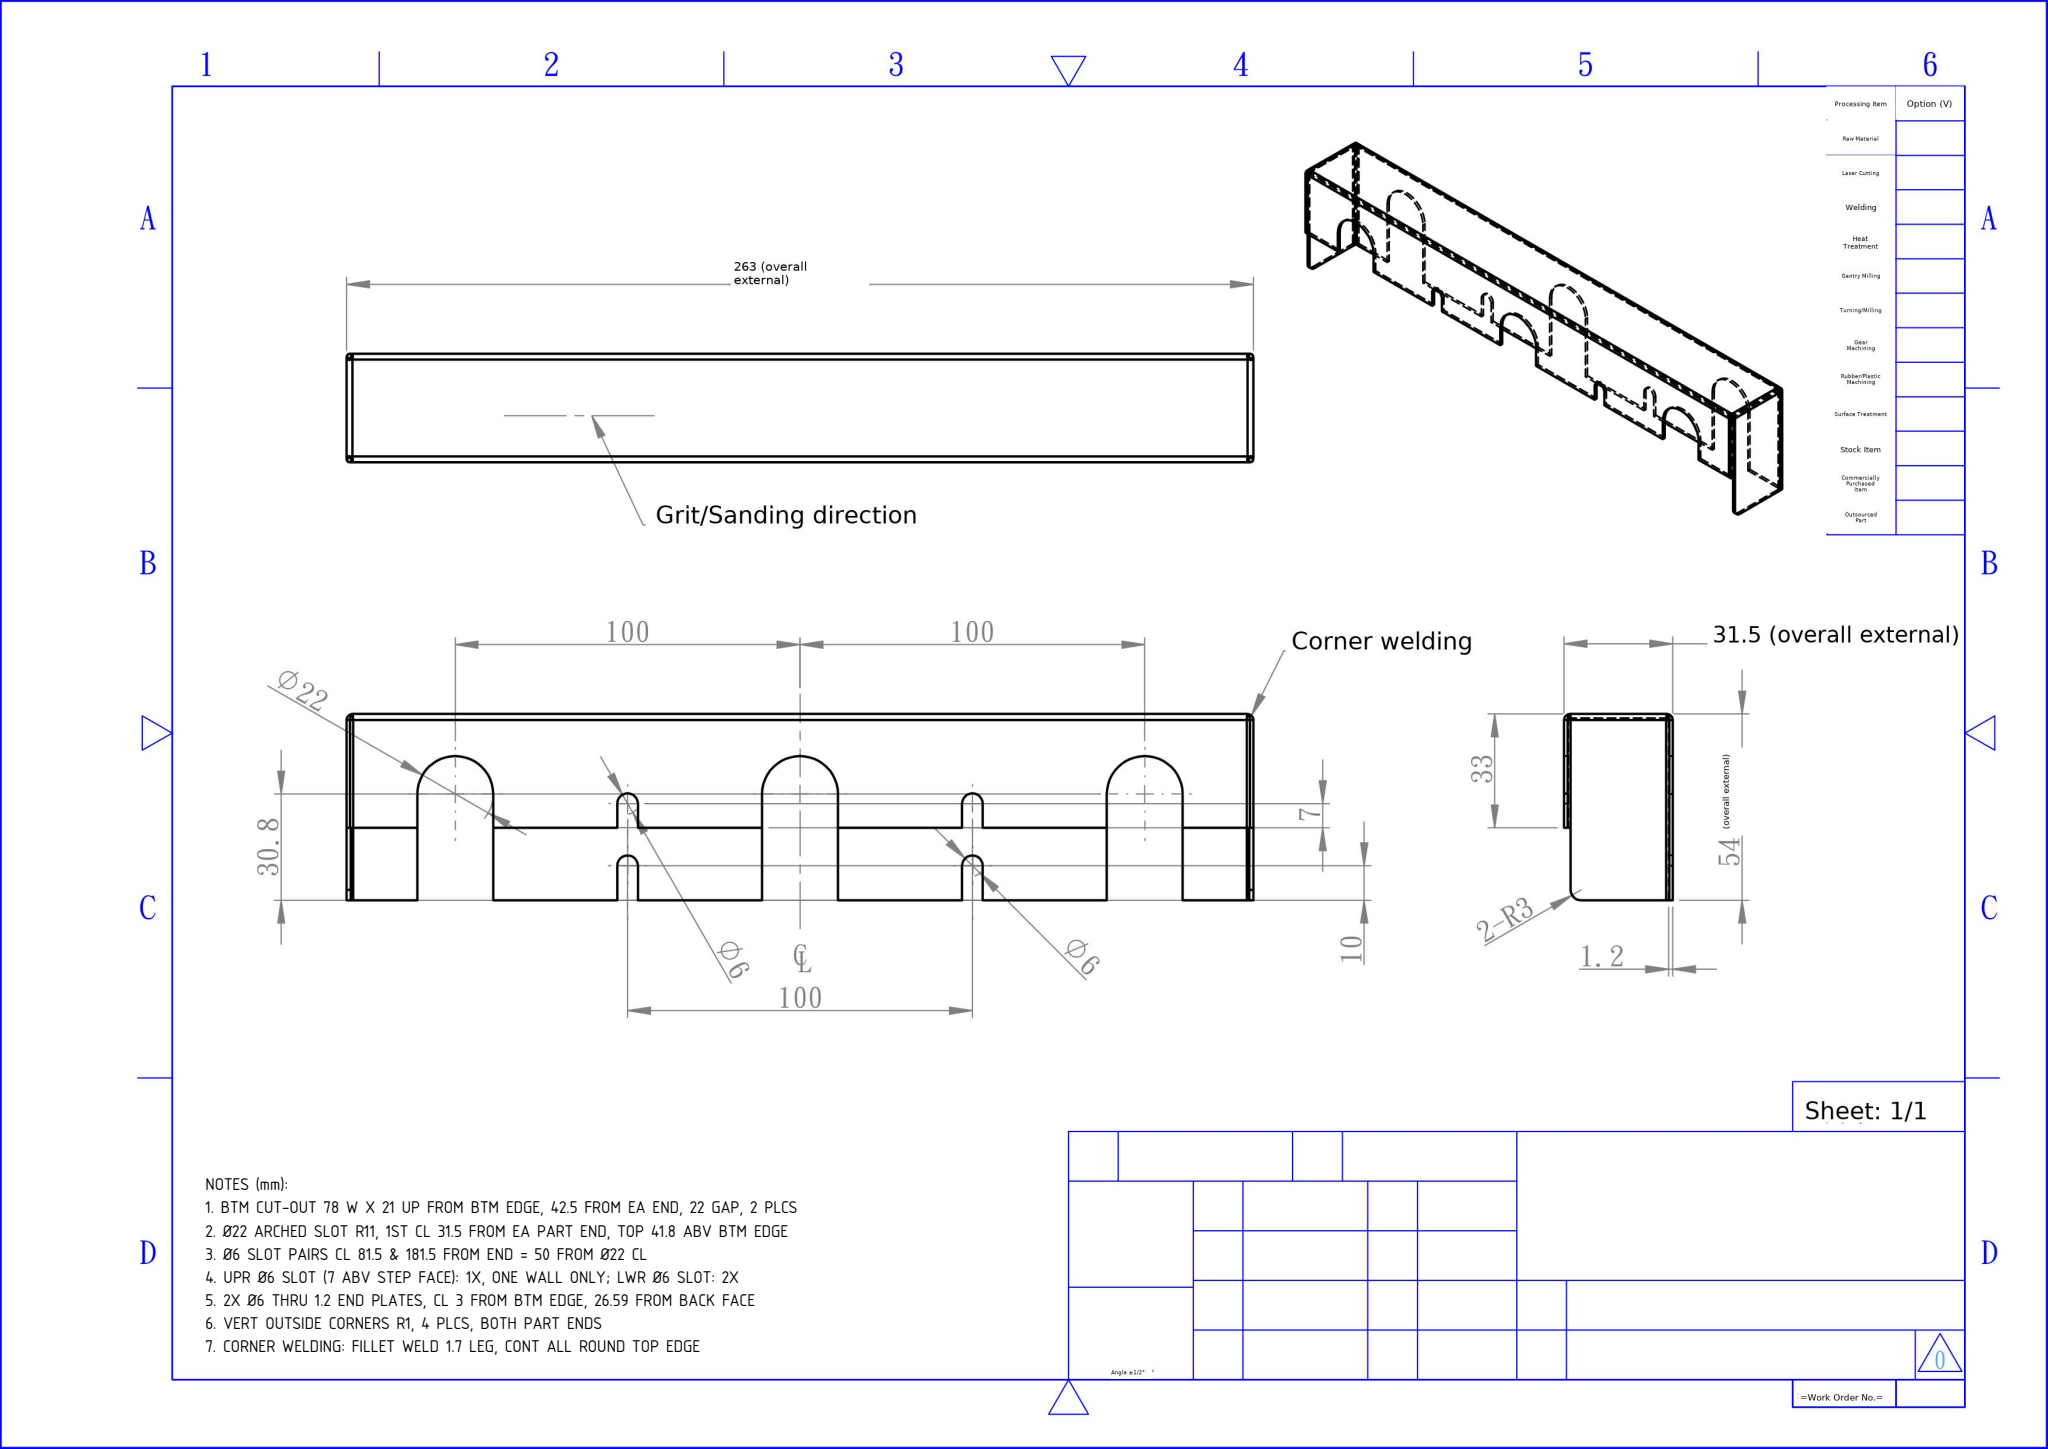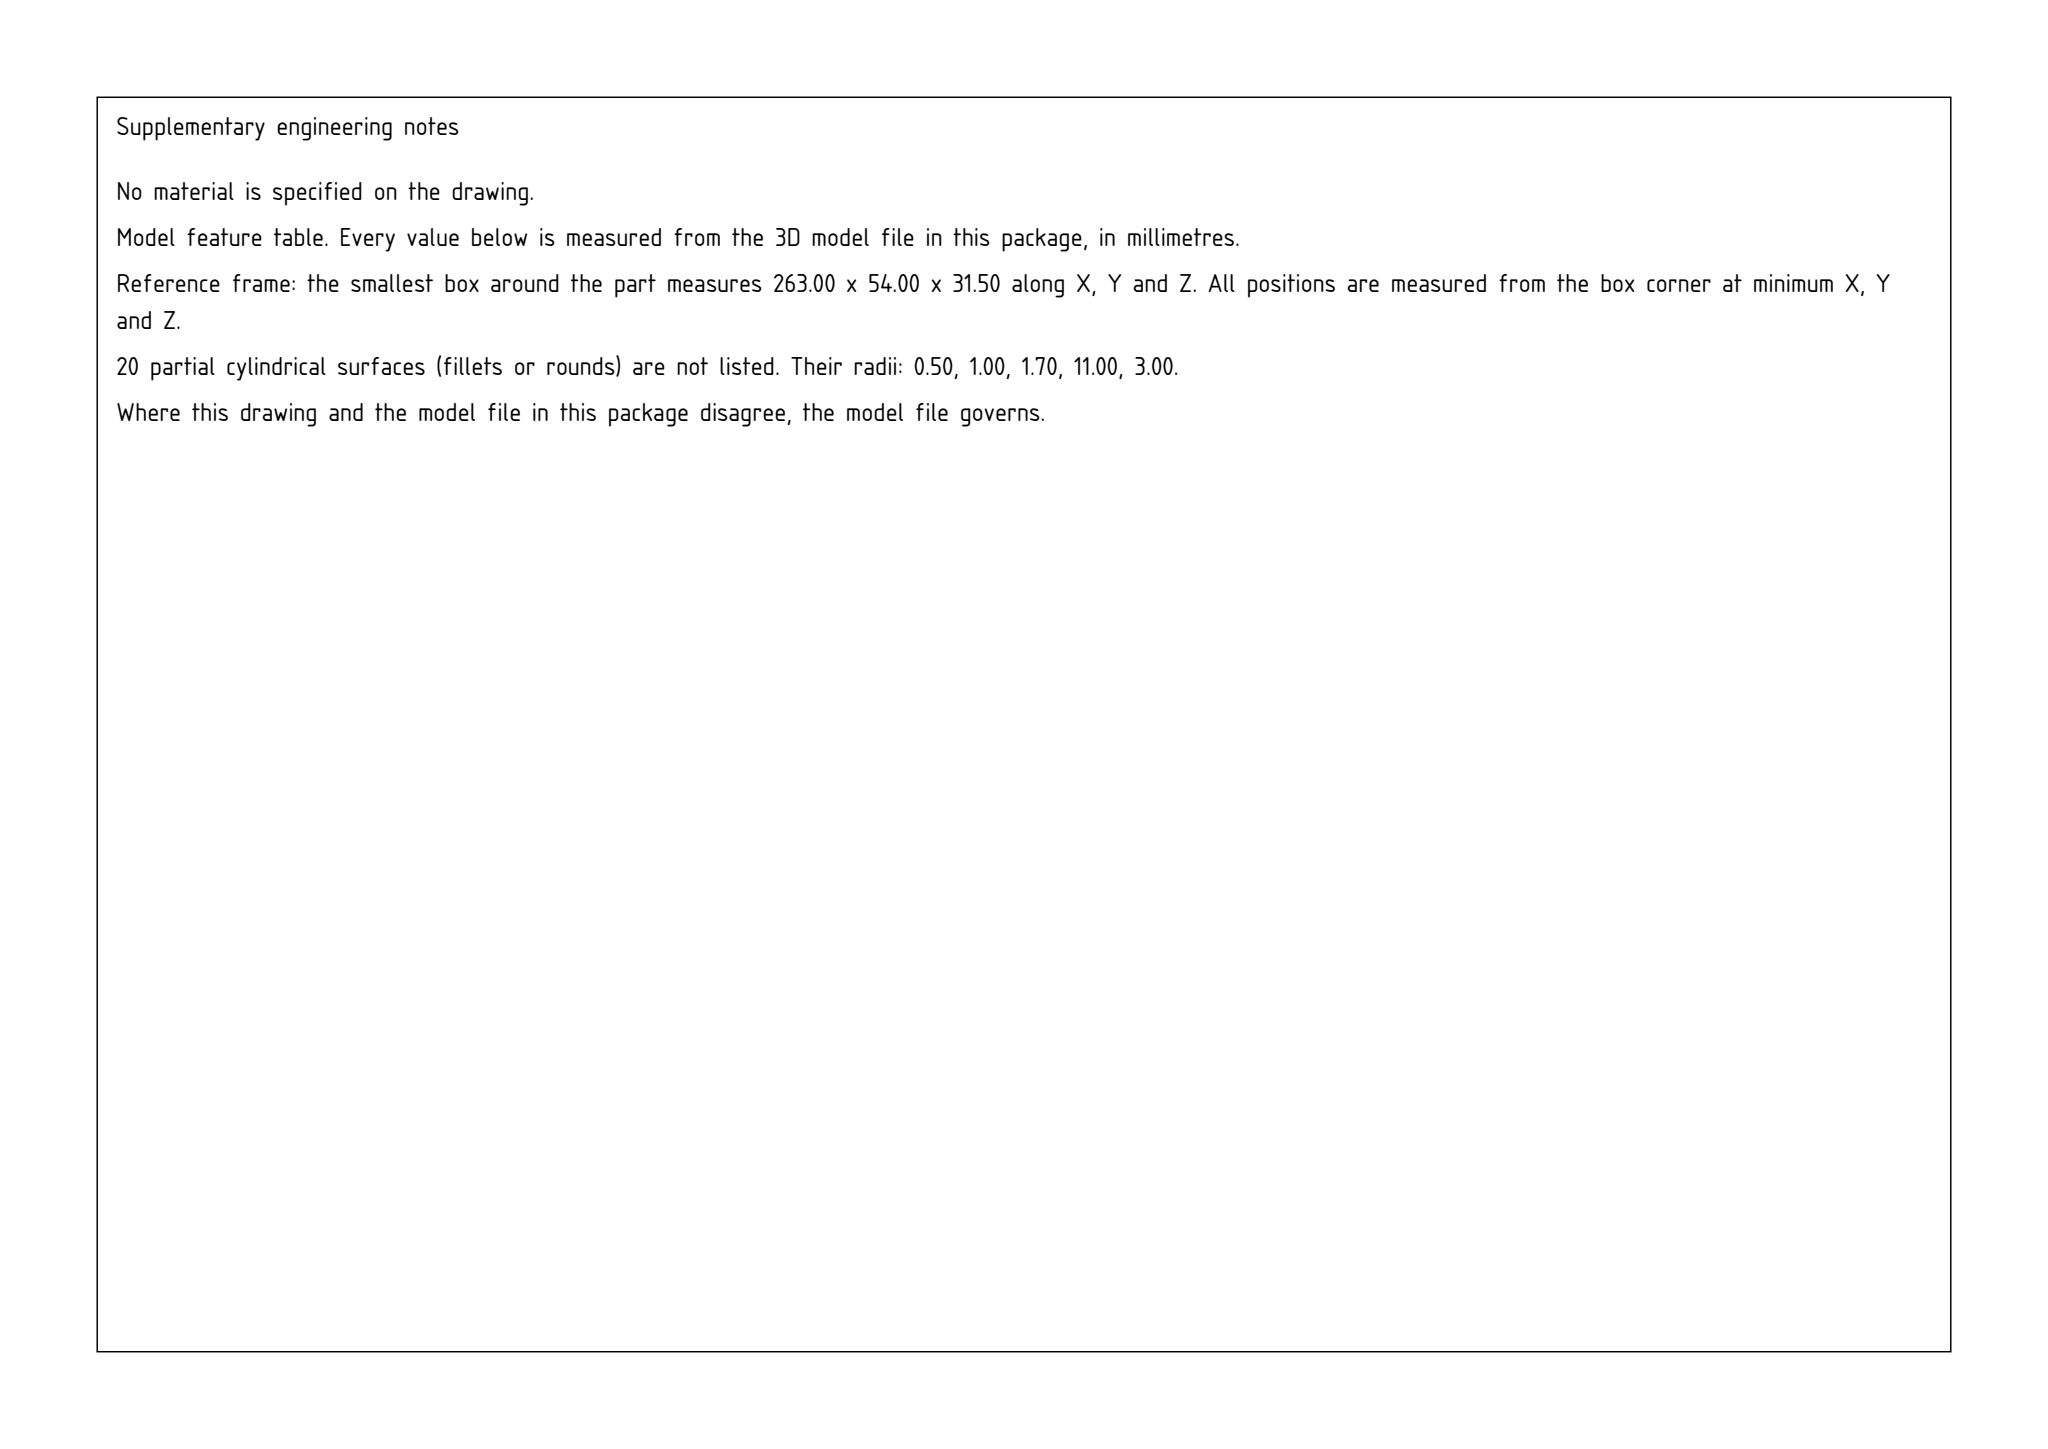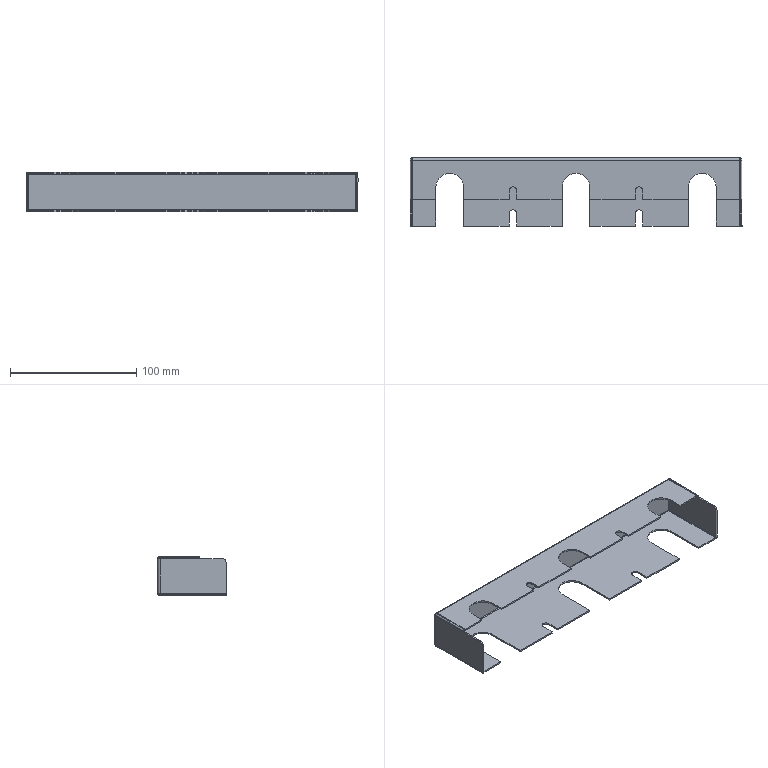Part | SolidWorks | mm | 1 solid | 118 faces | box 263 x 54 x 31.5 mm | volume 35024 mm3 | plane 66 | cylinder 32 | spline 20 | commonest cylinder face diameters 22 x12 6 x8 3.4 x4 1 x4 2 x4
Drawing notes:
BTM CUT-OUT 78 W X 21 UP FROM BTM EDGE, 42.5 FROM EA END, 22 GAP, 2 PLCS | from the solid: x-planes 42.5/120.5 and 142.5/220.5 (=78 ea), gap 142.5-120.5=22, 263-220.5=42.5; y plane 21 (8 faces) = cut floor
Ø22 ARCHED SLOT R11, 1ST CL 31.5 FROM EA PART END, TOP 41.8 ABV BTM EDGE | from the solid: Ø22 z-axis cyls at x=31.5/131.5/231.5, y=30.8; 263-231.5=31.5; 30.8+11=41.8
Ø6 SLOT PAIRS CL 81.5 & 181.5 FROM END = 50 FROM Ø22 CL | from the solid: Ø6 z-axis cyls at x=81.5 and 181.5; Ø22 CLs at 31.5/131.5/231.5
UPR Ø6 SLOT (7 ABV STEP FACE): 1X, ONE WALL ONLY; LWR Ø6 SLOT: 2X | from the solid: Ø6 z-cyl (81.5,28.0) count 1 and (181.5,28.0) count 1 vs (81.5,10.0) count 2 and (181.5,10.0) count 2
2X Ø6 THRU 1.2 END PLATES, CL 3 FROM BTM EDGE, 26.59 FROM BACK FACE | from the solid: cylinders [6.0,"x",[null,3.0,26.59],1.2,2] thru 1.2 thk end plates
VERT OUTSIDE CORNERS R1, 4 PLCS, BOTH PART ENDS | from the solid: Ø2 y-axis cyls at (x,z)=(1.0,1.0),(1.0,30.5),(262.0,1.0),(262.0,30.5)
CORNER WELDING: FILLET WELD 1.7 LEG, CONT ALL ROUND TOP EDGE | from the solid: weld bead cyls Ø3.4/Ø1.0 at y=52.3 (=54-1.7) along x at z=1.7 & 29.8 (L=259.6) and along z at x=1.7 & 261.3 (L=28.1)